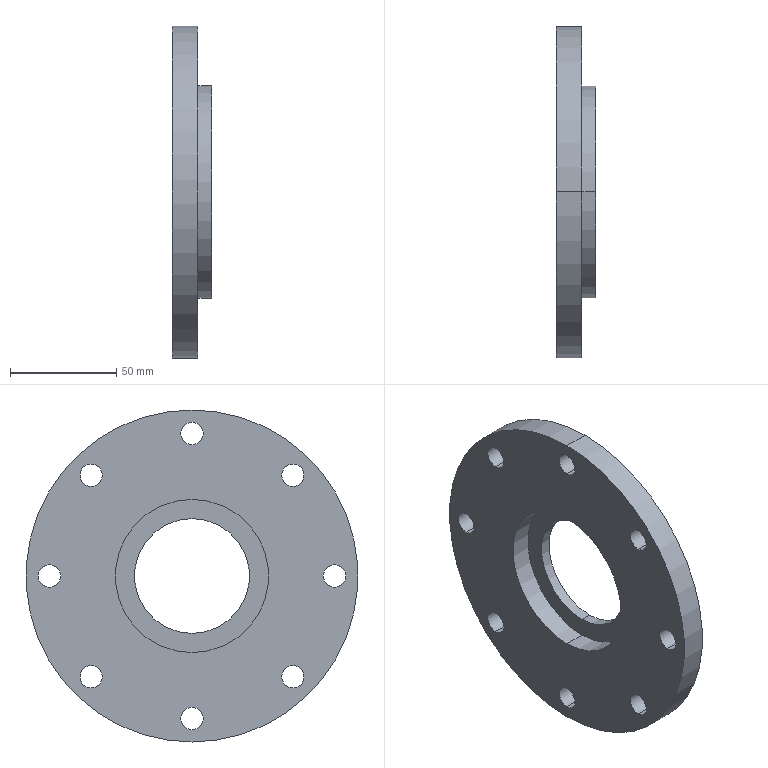Component | SolidWorks | UpperHousingAssembly-1_FlangeOnWormAxis-1 | 1 solid | 31 faces | box 18.5 x 156 x 156 mm | volume 196663 mm3 | cylinder 24 | plane 5 | cone 2 | commonest cylinder face diameters 10.5 x16 54 x2 100 x2 156 x2 72 x2
build123d program:
from build123d import *

# Parameters (mm, degrees)
SKETCH2_R          = 5.25
CUT_EXTRUDE1_DEPTH = 112.849
CIRPATTERN1_COUNT  = 8


with BuildPart() as part:
    # Sketch1 → Revolve1 (revolve)
    with BuildSketch(Plane.XY, mode=Mode.PRIVATE) as revolve1_sk:
        Polygon((0, 36), (0, 78), (12, 78), (12, 50), (18.5, 50), (18.5, 47), (15, 45), (15, 27), (10, 27), (10, 36), align=None)
    revolve(revolve1_sk.sketch.rotate(Axis((0, 0, 0), (1, 0, 0)), 90), axis=Axis((0, 0, 0), (1, 0, 0)))

    # Sketch2 → Cut-Extrude1 (cut, through all)
    with BuildSketch(Plane.ZY):
        with Locations((0, 67)):
            Circle(SKETCH2_R)
    cut_extrude1 = extrude(amount=-CUT_EXTRUDE1_DEPTH, mode=Mode.SUBTRACT)

    # CirPattern1: Cut-Extrude1 ×8 about axis
    cirpattern1_axis = Axis((0, 0, 0), (1, 0, 0))
    for i in range(1, CIRPATTERN1_COUNT):
        add(cut_extrude1.rotate(cirpattern1_axis, i * 360 / CIRPATTERN1_COUNT), mode=Mode.SUBTRACT)


solid = part.part

# Placed as in the assembly
solid = solid.moved(Location((719.83, 1408.591, 1694.217), (0, 0, 0)))
STEP:
#1=COLOUR_RGB('',0.7922,0.8196,0.9333);
#2=FILL_AREA_STYLE_COLOUR('',#1);
#3=FILL_AREA_STYLE('',(#2));
#4=SURFACE_STYLE_FILL_AREA(#3);
#5=SURFACE_SIDE_STYLE('',(#4));
#6=SURFACE_STYLE_USAGE(.BOTH.,#5);
#7=PRESENTATION_STYLE_ASSIGNMENT((#6));
#8=CARTESIAN_POINT('',(28.812,55.456,63.857));
#9=VERTEX_POINT('',#8);
#10=CARTESIAN_POINT('',(28.812,55.456,64.27));
#11=VERTEX_POINT('',#10);
#12=CARTESIAN_POINT('',(28.812,55.456,64.064));
#13=DIRECTION('',(-1.,0.,0.));
#14=DIRECTION('',(0.,0.,1.));
#15=AXIS2_PLACEMENT_3D('',#12,#13,#14);
#16=CIRCLE('',#15,0.2067);
#17=EDGE_CURVE('',#9,#11,#16,.T.);
#18=ORIENTED_EDGE('',*,*,#17,.F.);
#19=CARTESIAN_POINT('',(28.34,55.456,63.857));
#20=VERTEX_POINT('',#19);
#21=CARTESIAN_POINT('',(29.068,55.456,63.857));
#22=DIRECTION('',(-1.,0.,0.));
#23=VECTOR('',#22,39.37);
#24=LINE('',#21,#23);
#25=EDGE_CURVE('',#9,#20,#24,.T.);
#26=ORIENTED_EDGE('',*,*,#25,.T.);
#27=CARTESIAN_POINT('',(28.34,55.456,64.27));
#28=VERTEX_POINT('',#27);
#29=CARTESIAN_POINT('',(28.34,55.456,64.064));
#30=DIRECTION('',(-1.,0.,0.));
#31=DIRECTION('',(0.,1.,0.));
#32=AXIS2_PLACEMENT_3D('',#29,#30,#31);
#33=CIRCLE('',#32,0.2067);
#34=EDGE_CURVE('',#20,#28,#33,.T.);
#35=ORIENTED_EDGE('',*,*,#34,.T.);
#36=CARTESIAN_POINT('',(29.068,55.456,64.27));
#37=DIRECTION('',(-1.,0.,0.));
#38=VECTOR('',#37,39.37);
#39=LINE('',#36,#38);
#40=EDGE_CURVE('',#11,#28,#39,.T.);
#41=ORIENTED_EDGE('',*,*,#40,.F.);
#42=EDGE_LOOP('',(#18,#26,#35,#41));
#43=FACE_OUTER_BOUND('',#42,.T.);
#44=CARTESIAN_POINT('',(29.068,55.456,64.064));
#45=DIRECTION('',(-1.,0.,0.));
#46=DIRECTION('',(0.,0.,1.));
#47=AXIS2_PLACEMENT_3D('',#44,#45,#46);
#48=CYLINDRICAL_SURFACE('',#47,0.2067);
#49=ADVANCED_FACE('',(#43),#48,.F.);
#50=CARTESIAN_POINT('',(28.812,53.591,64.63));
#51=VERTEX_POINT('',#50);
#52=CARTESIAN_POINT('',(28.812,53.591,65.043));
#53=VERTEX_POINT('',#52);
#54=CARTESIAN_POINT('',(28.812,53.591,64.836));
#55=DIRECTION('',(-1.,0.,0.));
#56=DIRECTION('',(0.,0.,1.));
#57=AXIS2_PLACEMENT_3D('',#54,#55,#56);
#58=CIRCLE('',#57,0.2067);
#59=EDGE_CURVE('',#51,#53,#58,.T.);
#60=ORIENTED_EDGE('',*,*,#59,.F.);
#61=CARTESIAN_POINT('',(28.34,53.591,64.63));
#62=VERTEX_POINT('',#61);
#63=CARTESIAN_POINT('',(29.068,53.591,64.63));
#64=DIRECTION('',(-1.,0.,0.));
#65=VECTOR('',#64,39.37);
#66=LINE('',#63,#65);
#67=EDGE_CURVE('',#51,#62,#66,.T.);
#68=ORIENTED_EDGE('',*,*,#67,.T.);
#69=CARTESIAN_POINT('',(28.34,53.591,65.043));
#70=VERTEX_POINT('',#69);
#71=CARTESIAN_POINT('',(28.34,53.591,64.836));
#72=DIRECTION('',(-1.,0.,0.));
#73=DIRECTION('',(0.,0.7071,-0.7071));
#74=AXIS2_PLACEMENT_3D('',#71,#72,#73);
#75=CIRCLE('',#74,0.2067);
#76=EDGE_CURVE('',#62,#70,#75,.T.);
#77=ORIENTED_EDGE('',*,*,#76,.T.);
#78=CARTESIAN_POINT('',(29.068,53.591,65.043));
#79=DIRECTION('',(-1.,0.,0.));
#80=VECTOR('',#79,39.37);
#81=LINE('',#78,#80);
#82=EDGE_CURVE('',#53,#70,#81,.T.);
#83=ORIENTED_EDGE('',*,*,#82,.F.);
#84=EDGE_LOOP('',(#60,#68,#77,#83));
#85=FACE_OUTER_BOUND('',#84,.T.);
#86=CARTESIAN_POINT('',(29.068,53.591,64.836));
#87=DIRECTION('',(-1.,0.,0.));
#88=DIRECTION('',(0.,0.,1.));
#89=AXIS2_PLACEMENT_3D('',#86,#87,#88);
#90=CYLINDRICAL_SURFACE('',#89,0.2067);
#91=ADVANCED_FACE('',(#85),#90,.F.);
#92=CARTESIAN_POINT('',(28.812,52.819,66.495));
#93=VERTEX_POINT('',#92);
#94=CARTESIAN_POINT('',(28.812,52.819,66.908));
#95=VERTEX_POINT('',#94);
#96=CARTESIAN_POINT('',(28.812,52.819,66.701));
#97=DIRECTION('',(-1.,0.,0.));
#98=DIRECTION('',(0.,0.,1.));
#99=AXIS2_PLACEMENT_3D('',#96,#97,#98);
#100=CIRCLE('',#99,0.2067);
#101=EDGE_CURVE('',#93,#95,#100,.T.);
#102=ORIENTED_EDGE('',*,*,#101,.F.);
#103=CARTESIAN_POINT('',(28.34,52.819,66.495));
#104=VERTEX_POINT('',#103);
#105=CARTESIAN_POINT('',(29.068,52.819,66.495));
#106=DIRECTION('',(-1.,0.,0.));
#107=VECTOR('',#106,39.37);
#108=LINE('',#105,#107);
#109=EDGE_CURVE('',#93,#104,#108,.T.);
#110=ORIENTED_EDGE('',*,*,#109,.T.);
#111=CARTESIAN_POINT('',(28.34,52.819,66.908));
#112=VERTEX_POINT('',#111);
#113=CARTESIAN_POINT('',(28.34,52.819,66.701));
#114=DIRECTION('',(-1.,0.,0.));
#115=DIRECTION('',(0.,0.,-1.));
#116=AXIS2_PLACEMENT_3D('',#113,#114,#115);
#117=CIRCLE('',#116,0.2067);
#118=EDGE_CURVE('',#104,#112,#117,.T.);
#119=ORIENTED_EDGE('',*,*,#118,.T.);
#120=CARTESIAN_POINT('',(29.068,52.819,66.908));
#121=DIRECTION('',(-1.,0.,0.));
#122=VECTOR('',#121,39.37);
#123=LINE('',#120,#122);
#124=EDGE_CURVE('',#95,#112,#123,.T.);
#125=ORIENTED_EDGE('',*,*,#124,.F.);
#126=EDGE_LOOP('',(#102,#110,#119,#125));
#127=FACE_OUTER_BOUND('',#126,.T.);
#128=CARTESIAN_POINT('',(29.068,52.819,66.701));
#129=DIRECTION('',(-1.,0.,0.));
#130=DIRECTION('',(0.,0.,1.));
#131=AXIS2_PLACEMENT_3D('',#128,#129,#130);
#132=CYLINDRICAL_SURFACE('',#131,0.2067);
#133=ADVANCED_FACE('',(#127),#132,.F.);
#134=CARTESIAN_POINT('',(28.812,53.591,68.36));
#135=VERTEX_POINT('',#134);
#136=CARTESIAN_POINT('',(28.812,53.591,68.773));
#137=VERTEX_POINT('',#136);
#138=CARTESIAN_POINT('',(28.812,53.591,68.567));
#139=DIRECTION('',(-1.,0.,0.));
#140=DIRECTION('',(0.,0.,1.));
#141=AXIS2_PLACEMENT_3D('',#138,#139,#140);
#142=CIRCLE('',#141,0.2067);
#143=EDGE_CURVE('',#135,#137,#142,.T.);
#144=ORIENTED_EDGE('',*,*,#143,.F.);
#145=CARTESIAN_POINT('',(28.34,53.591,68.36));
#146=VERTEX_POINT('',#145);
#147=CARTESIAN_POINT('',(29.068,53.591,68.36));
#148=DIRECTION('',(-1.,0.,0.));
#149=VECTOR('',#148,39.37);
#150=LINE('',#147,#149);
#151=EDGE_CURVE('',#135,#146,#150,.T.);
#152=ORIENTED_EDGE('',*,*,#151,.T.);
#153=CARTESIAN_POINT('',(28.34,53.591,68.773));
#154=VERTEX_POINT('',#153);
#155=CARTESIAN_POINT('',(28.34,53.591,68.567));
#156=DIRECTION('',(-1.,0.,0.));
#157=DIRECTION('',(0.,-0.7071,-0.7071));
#158=AXIS2_PLACEMENT_3D('',#155,#156,#157);
#159=CIRCLE('',#158,0.2067);
#160=EDGE_CURVE('',#146,#154,#159,.T.);
#161=ORIENTED_EDGE('',*,*,#160,.T.);
#162=CARTESIAN_POINT('',(29.068,53.591,68.773));
#163=DIRECTION('',(-1.,0.,0.));
#164=VECTOR('',#163,39.37);
#165=LINE('',#162,#164);
#166=EDGE_CURVE('',#137,#154,#165,.T.);
#167=ORIENTED_EDGE('',*,*,#166,.F.);
#168=EDGE_LOOP('',(#144,#152,#161,#167));
#169=FACE_OUTER_BOUND('',#168,.T.);
#170=CARTESIAN_POINT('',(29.068,53.591,68.567));
#171=DIRECTION('',(-1.,0.,0.));
#172=DIRECTION('',(0.,0.,1.));
#173=AXIS2_PLACEMENT_3D('',#170,#171,#172);
#174=CYLINDRICAL_SURFACE('',#173,0.2067);
#175=ADVANCED_FACE('',(#169),#174,.F.);
#176=CARTESIAN_POINT('',(28.812,55.456,69.133));
#177=VERTEX_POINT('',#176);
#178=CARTESIAN_POINT('',(28.812,55.456,69.546));
#179=VERTEX_POINT('',#178);
#180=CARTESIAN_POINT('',(28.812,55.456,69.339));
#181=DIRECTION('',(-1.,0.,0.));
#182=DIRECTION('',(0.,0.,1.));
#183=AXIS2_PLACEMENT_3D('',#180,#181,#182);
#184=CIRCLE('',#183,0.2067);
#185=EDGE_CURVE('',#177,#179,#184,.T.);
#186=ORIENTED_EDGE('',*,*,#185,.F.);
#187=CARTESIAN_POINT('',(28.34,55.456,69.133));
#188=VERTEX_POINT('',#187);
#189=CARTESIAN_POINT('',(29.068,55.456,69.133));
#190=DIRECTION('',(-1.,0.,0.));
#191=VECTOR('',#190,39.37);
#192=LINE('',#189,#191);
#193=EDGE_CURVE('',#177,#188,#192,.T.);
#194=ORIENTED_EDGE('',*,*,#193,.T.);
#195=CARTESIAN_POINT('',(28.34,55.456,69.546));
#196=VERTEX_POINT('',#195);
#197=CARTESIAN_POINT('',(28.34,55.456,69.339));
#198=DIRECTION('',(-1.,0.,0.));
#199=DIRECTION('',(0.,-1.,0.));
#200=AXIS2_PLACEMENT_3D('',#197,#198,#199);
#201=CIRCLE('',#200,0.2067);
#202=EDGE_CURVE('',#188,#196,#201,.T.);
#203=ORIENTED_EDGE('',*,*,#202,.T.);
#204=CARTESIAN_POINT('',(29.068,55.456,69.546));
#205=DIRECTION('',(-1.,0.,0.));
#206=VECTOR('',#205,39.37);
#207=LINE('',#204,#206);
#208=EDGE_CURVE('',#179,#196,#207,.T.);
#209=ORIENTED_EDGE('',*,*,#208,.F.);
#210=EDGE_LOOP('',(#186,#194,#203,#209));
#211=FACE_OUTER_BOUND('',#210,.T.);
#212=CARTESIAN_POINT('',(29.068,55.456,69.339));
#213=DIRECTION('',(-1.,0.,0.));
#214=DIRECTION('',(0.,0.,1.));
#215=AXIS2_PLACEMENT_3D('',#212,#213,#214);
#216=CYLINDRICAL_SURFACE('',#215,0.2067);
#217=ADVANCED_FACE('',(#211),#216,.F.);
#218=CARTESIAN_POINT('',(28.812,57.322,68.36));
#219=VERTEX_POINT('',#218);
#220=CARTESIAN_POINT('',(28.812,57.322,68.773));
#221=VERTEX_POINT('',#220);
#222=CARTESIAN_POINT('',(28.812,57.322,68.567));
#223=DIRECTION('',(-1.,0.,0.));
#224=DIRECTION('',(0.,0.,1.));
#225=AXIS2_PLACEMENT_3D('',#222,#223,#224);
#226=CIRCLE('',#225,0.2067);
#227=EDGE_CURVE('',#219,#221,#226,.T.);
#228=ORIENTED_EDGE('',*,*,#227,.F.);
#229=CARTESIAN_POINT('',(28.34,57.322,68.36));
#230=VERTEX_POINT('',#229);
#231=CARTESIAN_POINT('',(29.068,57.322,68.36));
#232=DIRECTION('',(-1.,0.,0.));
#233=VECTOR('',#232,39.37);
#234=LINE('',#231,#233);
#235=EDGE_CURVE('',#219,#230,#234,.T.);
#236=ORIENTED_EDGE('',*,*,#235,.T.);
#237=CARTESIAN_POINT('',(28.34,57.322,68.773));
#238=VERTEX_POINT('',#237);
#239=CARTESIAN_POINT('',(28.34,57.322,68.567));
#240=DIRECTION('',(-1.,0.,0.));
#241=DIRECTION('',(0.,-0.7071,0.7071));
#242=AXIS2_PLACEMENT_3D('',#239,#240,#241);
#243=CIRCLE('',#242,0.2067);
#244=EDGE_CURVE('',#230,#238,#243,.T.);
#245=ORIENTED_EDGE('',*,*,#244,.T.);
#246=CARTESIAN_POINT('',(29.068,57.322,68.773));
#247=DIRECTION('',(-1.,0.,0.));
#248=VECTOR('',#247,39.37);
#249=LINE('',#246,#248);
#250=EDGE_CURVE('',#221,#238,#249,.T.);
#251=ORIENTED_EDGE('',*,*,#250,.F.);
#252=EDGE_LOOP('',(#228,#236,#245,#251));
#253=FACE_OUTER_BOUND('',#252,.T.);
#254=CARTESIAN_POINT('',(29.068,57.322,68.567));
#255=DIRECTION('',(-1.,0.,0.));
#256=DIRECTION('',(0.,0.,1.));
#257=AXIS2_PLACEMENT_3D('',#254,#255,#256);
#258=CYLINDRICAL_SURFACE('',#257,0.2067);
#259=ADVANCED_FACE('',(#253),#258,.F.);
#260=CARTESIAN_POINT('',(28.812,57.322,64.63));
#261=VERTEX_POINT('',#260);
#262=CARTESIAN_POINT('',(28.812,57.322,65.043));
#263=VERTEX_POINT('',#262);
#264=CARTESIAN_POINT('',(28.812,57.322,64.836));
#265=DIRECTION('',(-1.,0.,0.));
#266=DIRECTION('',(0.,0.,1.));
#267=AXIS2_PLACEMENT_3D('',#264,#265,#266);
#268=CIRCLE('',#267,0.2067);
#269=EDGE_CURVE('',#261,#263,#268,.T.);
#270=ORIENTED_EDGE('',*,*,#269,.F.);
#271=CARTESIAN_POINT('',(28.34,57.322,64.63));
#272=VERTEX_POINT('',#271);
#273=CARTESIAN_POINT('',(29.068,57.322,64.63));
#274=DIRECTION('',(-1.,0.,0.));
#275=VECTOR('',#274,39.37);
#276=LINE('',#273,#275);
#277=EDGE_CURVE('',#261,#272,#276,.T.);
#278=ORIENTED_EDGE('',*,*,#277,.T.);
#279=CARTESIAN_POINT('',(28.34,57.322,65.043));
#280=VERTEX_POINT('',#279);
#281=CARTESIAN_POINT('',(28.34,57.322,64.836));
#282=DIRECTION('',(-1.,0.,0.));
#283=DIRECTION('',(0.,0.7071,0.7071));
#284=AXIS2_PLACEMENT_3D('',#281,#282,#283);
#285=CIRCLE('',#284,0.2067);
#286=EDGE_CURVE('',#272,#280,#285,.T.);
#287=ORIENTED_EDGE('',*,*,#286,.T.);
#288=CARTESIAN_POINT('',(29.068,57.322,65.043));
#289=DIRECTION('',(-1.,0.,0.));
#290=VECTOR('',#289,39.37);
#291=LINE('',#288,#290);
#292=EDGE_CURVE('',#263,#280,#291,.T.);
#293=ORIENTED_EDGE('',*,*,#292,.F.);
#294=EDGE_LOOP('',(#270,#278,#287,#293));
#295=FACE_OUTER_BOUND('',#294,.T.);
#296=CARTESIAN_POINT('',(29.068,57.322,64.836));
#297=DIRECTION('',(-1.,0.,0.));
#298=DIRECTION('',(0.,0.,1.));
#299=AXIS2_PLACEMENT_3D('',#296,#297,#298);
#300=CYLINDRICAL_SURFACE('',#299,0.2067);
#301=ADVANCED_FACE('',(#295),#300,.F.);
#302=CARTESIAN_POINT('',(28.812,58.094,66.495));
#303=VERTEX_POINT('',#302);
#304=CARTESIAN_POINT('',(28.812,58.094,66.908));
#305=VERTEX_POINT('',#304);
#306=CARTESIAN_POINT('',(28.812,58.094,66.701));
#307=DIRECTION('',(-1.,0.,0.));
#308=DIRECTION('',(0.,0.,1.));
#309=AXIS2_PLACEMENT_3D('',#306,#307,#308);
#310=CIRCLE('',#309,0.2067);
#311=EDGE_CURVE('',#303,#305,#310,.T.);
#312=ORIENTED_EDGE('',*,*,#311,.F.);
#313=CARTESIAN_POINT('',(28.34,58.094,66.495));
#314=VERTEX_POINT('',#313);
#315=CARTESIAN_POINT('',(29.068,58.094,66.495));
#316=DIRECTION('',(-1.,0.,0.));
#317=VECTOR('',#316,39.37);
#318=LINE('',#315,#317);
#319=EDGE_CURVE('',#303,#314,#318,.T.);
#320=ORIENTED_EDGE('',*,*,#319,.T.);
#321=CARTESIAN_POINT('',(28.34,58.094,66.908));
#322=VERTEX_POINT('',#321);
#323=CARTESIAN_POINT('',(28.34,58.094,66.701));
#324=DIRECTION('',(-1.,0.,0.));
#325=DIRECTION('',(0.,0.,1.));
#326=AXIS2_PLACEMENT_3D('',#323,#324,#325);
#327=CIRCLE('',#326,0.2067);
#328=EDGE_CURVE('',#314,#322,#327,.T.);
#329=ORIENTED_EDGE('',*,*,#328,.T.);
#330=CARTESIAN_POINT('',(29.068,58.094,66.908));
#331=DIRECTION('',(-1.,0.,0.));
#332=VECTOR('',#331,39.37);
#333=LINE('',#330,#332);
#334=EDGE_CURVE('',#305,#322,#333,.T.);
#335=ORIENTED_EDGE('',*,*,#334,.F.);
#336=EDGE_LOOP('',(#312,#320,#329,#335));
#337=FACE_OUTER_BOUND('',#336,.T.);
#338=CARTESIAN_POINT('',(29.068,58.094,66.701));
#339=DIRECTION('',(-1.,0.,0.));
#340=DIRECTION('',(0.,0.,1.));
#341=AXIS2_PLACEMENT_3D('',#338,#339,#340);
#342=CYLINDRICAL_SURFACE('',#341,0.2067);
#343=ADVANCED_FACE('',(#337),#342,.F.);
#344=CARTESIAN_POINT('',(28.93,55.456,65.638));
#345=VERTEX_POINT('',#344);
#346=CARTESIAN_POINT('',(28.93,55.456,67.764));
#347=VERTEX_POINT('',#346);
#348=CARTESIAN_POINT('',(28.93,55.456,66.701));
#349=DIRECTION('',(-1.,0.,0.));
#350=DIRECTION('',(0.,0.,1.));
#351=AXIS2_PLACEMENT_3D('',#348,#349,#350);
#352=CIRCLE('',#351,1.063);
#353=EDGE_CURVE('',#345,#347,#352,.T.);
#354=ORIENTED_EDGE('',*,*,#353,.F.);
#355=CARTESIAN_POINT('',(28.733,55.456,65.638));
#356=VERTEX_POINT('',#355);
#357=CARTESIAN_POINT('',(28.34,55.456,65.638));
#358=DIRECTION('',(-1.,0.,0.));
#359=VECTOR('',#358,39.37);
#360=LINE('',#357,#359);
#361=EDGE_CURVE('',#345,#356,#360,.T.);
#362=ORIENTED_EDGE('',*,*,#361,.T.);
#363=CARTESIAN_POINT('',(28.733,55.456,67.764));
#364=VERTEX_POINT('',#363);
#365=CARTESIAN_POINT('',(28.733,55.456,66.701));
#366=DIRECTION('',(-1.,0.,0.));
#367=DIRECTION('',(0.,0.,1.));
#368=AXIS2_PLACEMENT_3D('',#365,#366,#367);
#369=CIRCLE('',#368,1.063);
#370=EDGE_CURVE('',#356,#364,#369,.T.);
#371=ORIENTED_EDGE('',*,*,#370,.T.);
#372=CARTESIAN_POINT('',(28.34,55.456,67.764));
#373=DIRECTION('',(-1.,0.,0.));
#374=VECTOR('',#373,39.37);
#375=LINE('',#372,#374);
#376=EDGE_CURVE('',#347,#364,#375,.T.);
#377=ORIENTED_EDGE('',*,*,#376,.F.);
#378=EDGE_LOOP('',(#354,#362,#371,#377));
#379=FACE_OUTER_BOUND('',#378,.T.);
#380=CARTESIAN_POINT('',(28.34,55.456,66.701));
#381=DIRECTION('',(-1.,0.,0.));
#382=DIRECTION('',(0.,0.,1.));
#383=AXIS2_PLACEMENT_3D('',#380,#381,#382);
#384=CYLINDRICAL_SURFACE('',#383,1.063);
#385=ADVANCED_FACE('',(#379),#384,.F.);
#386=CARTESIAN_POINT('',(28.93,55.456,64.93));
#387=VERTEX_POINT('',#386);
#388=CARTESIAN_POINT('',(28.93,55.456,68.473));
#389=VERTEX_POINT('',#388);
#390=CARTESIAN_POINT('',(28.93,55.456,66.701));
#391=DIRECTION('',(-1.,0.,0.));
#392=DIRECTION('',(0.,0.,1.));
#393=AXIS2_PLACEMENT_3D('',#390,#391,#392);
#394=CIRCLE('',#393,1.772);
#395=EDGE_CURVE('',#387,#389,#394,.T.);
#396=ORIENTED_EDGE('',*,*,#395,.T.);
#397=CARTESIAN_POINT('',(29.068,55.456,68.552));
#398=VERTEX_POINT('',#397);
#399=CARTESIAN_POINT('',(28.93,55.456,68.473));
#400=DIRECTION('',(0.8682,0.,0.4961));
#401=VECTOR('',#400,39.37);
#402=LINE('',#399,#401);
#403=EDGE_CURVE('',#389,#398,#402,.T.);
#404=ORIENTED_EDGE('',*,*,#403,.T.);
#405=CARTESIAN_POINT('',(29.068,55.456,64.851));
#406=VERTEX_POINT('',#405);
#407=CARTESIAN_POINT('',(29.068,55.456,66.701));
#408=DIRECTION('',(-1.,0.,0.));
#409=DIRECTION('',(0.,0.,1.));
#410=AXIS2_PLACEMENT_3D('',#407,#408,#409);
#411=CIRCLE('',#410,1.85);
#412=EDGE_CURVE('',#406,#398,#411,.T.);
#413=ORIENTED_EDGE('',*,*,#412,.F.);
#414=CARTESIAN_POINT('',(28.93,55.456,64.93));
#415=DIRECTION('',(0.8682,0.,-0.4961));
#416=VECTOR('',#415,39.37);
#417=LINE('',#414,#416);
#418=EDGE_CURVE('',#387,#406,#417,.T.);
#419=ORIENTED_EDGE('',*,*,#418,.F.);
#420=EDGE_LOOP('',(#396,#404,#413,#419));
#421=FACE_OUTER_BOUND('',#420,.T.);
#422=CARTESIAN_POINT('',(28.93,55.456,66.701));
#423=DIRECTION('',(1.,0.,0.));
#424=DIRECTION('',(0.,0.,-1.));
#425=AXIS2_PLACEMENT_3D('',#422,#423,#424);
#426=CONICAL_SURFACE('',#425,1.772,0.5191);
#427=ADVANCED_FACE('',(#421),#426,.F.);
#428=CARTESIAN_POINT('',(29.068,55.456,68.67));
#429=VERTEX_POINT('',#428);
#430=CARTESIAN_POINT('',(29.068,55.456,64.733));
#431=VERTEX_POINT('',#430);
#432=CARTESIAN_POINT('',(29.068,55.456,66.701));
#433=DIRECTION('',(-1.,0.,0.));
#434=DIRECTION('',(0.,0.,1.));
#435=AXIS2_PLACEMENT_3D('',#432,#433,#434);
#436=CIRCLE('',#435,1.969);
#437=EDGE_CURVE('',#429,#431,#436,.T.);
#438=ORIENTED_EDGE('',*,*,#437,.T.);
#439=CARTESIAN_POINT('',(28.812,55.456,64.733));
#440=VERTEX_POINT('',#439);
#441=CARTESIAN_POINT('',(28.34,55.456,64.733));
#442=DIRECTION('',(-1.,0.,0.));
#443=VECTOR('',#442,39.37);
#444=LINE('',#441,#443);
#445=EDGE_CURVE('',#431,#440,#444,.T.);
#446=ORIENTED_EDGE('',*,*,#445,.T.);
#447=CARTESIAN_POINT('',(28.812,55.456,68.67));
#448=VERTEX_POINT('',#447);
#449=CARTESIAN_POINT('',(28.812,55.456,66.701));
#450=DIRECTION('',(-1.,0.,0.));
#451=DIRECTION('',(0.,0.,1.));
#452=AXIS2_PLACEMENT_3D('',#449,#450,#451);
#453=CIRCLE('',#452,1.969);
#454=EDGE_CURVE('',#448,#440,#453,.T.);
#455=ORIENTED_EDGE('',*,*,#454,.F.);
#456=CARTESIAN_POINT('',(28.34,55.456,68.67));
#457=DIRECTION('',(-1.,0.,0.));
#458=VECTOR('',#457,39.37);
#459=LINE('',#456,#458);
#460=EDGE_CURVE('',#429,#448,#459,.T.);
#461=ORIENTED_EDGE('',*,*,#460,.F.);
#462=EDGE_LOOP('',(#438,#446,#455,#461));
#463=FACE_OUTER_BOUND('',#462,.T.);
#464=CARTESIAN_POINT('',(28.34,55.456,66.701));
#465=DIRECTION('',(-1.,0.,0.));
#466=DIRECTION('',(0.,0.,1.));
#467=AXIS2_PLACEMENT_3D('',#464,#465,#466);
#468=CYLINDRICAL_SURFACE('',#467,1.969);
#469=ADVANCED_FACE('',(#463),#468,.T.);
#470=CARTESIAN_POINT('',(28.812,55.456,69.772));
#471=VERTEX_POINT('',#470);
#472=CARTESIAN_POINT('',(28.812,55.456,63.631));
#473=VERTEX_POINT('',#472);
#474=CARTESIAN_POINT('',(28.812,55.456,66.701));
#475=DIRECTION('',(-1.,0.,0.));
#476=DIRECTION('',(0.,0.,1.));
#477=AXIS2_PLACEMENT_3D('',#474,#475,#476);
#478=CIRCLE('',#477,3.071);
#479=EDGE_CURVE('',#471,#473,#478,.T.);
#480=ORIENTED_EDGE('',*,*,#479,.T.);
#481=CARTESIAN_POINT('',(28.34,55.456,63.631));
#482=VERTEX_POINT('',#481);
#483=CARTESIAN_POINT('',(28.34,55.456,63.631));
#484=DIRECTION('',(-1.,0.,0.));
#485=VECTOR('',#484,39.37);
#486=LINE('',#483,#485);
#487=EDGE_CURVE('',#473,#482,#486,.T.);
#488=ORIENTED_EDGE('',*,*,#487,.T.);
#489=CARTESIAN_POINT('',(28.34,55.456,69.772));
#490=VERTEX_POINT('',#489);
#491=CARTESIAN_POINT('',(28.34,55.456,66.701));
#492=DIRECTION('',(-1.,0.,0.));
#493=DIRECTION('',(0.,0.,1.));
#494=AXIS2_PLACEMENT_3D('',#491,#492,#493);
#495=CIRCLE('',#494,3.071);
#496=EDGE_CURVE('',#490,#482,#495,.T.);
#497=ORIENTED_EDGE('',*,*,#496,.F.);
#498=CARTESIAN_POINT('',(28.34,55.456,69.772));
#499=DIRECTION('',(-1.,0.,0.));
#500=VECTOR('',#499,39.37);
#501=LINE('',#498,#500);
#502=EDGE_CURVE('',#471,#490,#501,.T.);
#503=ORIENTED_EDGE('',*,*,#502,.F.);
#504=EDGE_LOOP('',(#480,#488,#497,#503));
#505=FACE_OUTER_BOUND('',#504,.T.);
#506=CARTESIAN_POINT('',(28.34,55.456,66.701));
#507=DIRECTION('',(-1.,0.,0.));
#508=DIRECTION('',(0.,0.,1.));
#509=AXIS2_PLACEMENT_3D('',#506,#507,#508);
#510=CYLINDRICAL_SURFACE('',#509,3.071);
#511=ADVANCED_FACE('',(#505),#510,.T.);
#512=CARTESIAN_POINT('',(28.733,55.456,65.284));
#513=VERTEX_POINT('',#512);
#514=CARTESIAN_POINT('',(28.733,55.456,68.119));
#515=VERTEX_POINT('',#514);
#516=CARTESIAN_POINT('',(28.733,55.456,66.701));
#517=DIRECTION('',(-1.,0.,0.));
#518=DIRECTION('',(0.,0.,1.));
#519=AXIS2_PLACEMENT_3D('',#516,#517,#518);
#520=CIRCLE('',#519,1.417);
#521=EDGE_CURVE('',#513,#515,#520,.T.);
#522=ORIENTED_EDGE('',*,*,#521,.F.);
#523=CARTESIAN_POINT('',(28.34,55.456,65.284));
#524=VERTEX_POINT('',#523);
#525=CARTESIAN_POINT('',(28.34,55.456,65.284));
#526=DIRECTION('',(-1.,0.,0.));
#527=VECTOR('',#526,39.37);
#528=LINE('',#525,#527);
#529=EDGE_CURVE('',#513,#524,#528,.T.);
#530=ORIENTED_EDGE('',*,*,#529,.T.);
#531=CARTESIAN_POINT('',(28.34,55.456,68.119));
#532=VERTEX_POINT('',#531);
#533=CARTESIAN_POINT('',(28.34,55.456,66.701));
#534=DIRECTION('',(-1.,0.,0.));
#535=DIRECTION('',(0.,0.,1.));
#536=AXIS2_PLACEMENT_3D('',#533,#534,#535);
#537=CIRCLE('',#536,1.417);
#538=EDGE_CURVE('',#524,#532,#537,.T.);
#539=ORIENTED_EDGE('',*,*,#538,.T.);
#540=CARTESIAN_POINT('',(28.34,55.456,68.119));
#541=DIRECTION('',(-1.,0.,0.));
#542=VECTOR('',#541,39.37);
#543=LINE('',#540,#542);
#544=EDGE_CURVE('',#515,#532,#543,.T.);
#545=ORIENTED_EDGE('',*,*,#544,.F.);
#546=EDGE_LOOP('',(#522,#530,#539,#545));
#547=FACE_OUTER_BOUND('',#546,.T.);
#548=CARTESIAN_POINT('',(28.34,55.456,66.701));
#549=DIRECTION('',(-1.,0.,0.));
#550=DIRECTION('',(0.,0.,1.));
#551=AXIS2_PLACEMENT_3D('',#548,#549,#550);
#552=CYLINDRICAL_SURFACE('',#551,1.417);
#553=ADVANCED_FACE('',(#547),#552,.F.);
#554=ORIENTED_EDGE('',*,*,#529,.F.);
#555=CARTESIAN_POINT('',(28.733,55.456,66.701));
#556=DIRECTION('',(-1.,0.,0.));
#557=DIRECTION('',(0.,0.,1.));
#558=AXIS2_PLACEMENT_3D('',#555,#556,#557);
#559=CIRCLE('',#558,1.417);
#560=EDGE_CURVE('',#515,#513,#559,.T.);
#561=ORIENTED_EDGE('',*,*,#560,.F.);
#562=ORIENTED_EDGE('',*,*,#544,.T.);
#563=CARTESIAN_POINT('',(28.34,55.456,66.701));
#564=DIRECTION('',(-1.,0.,0.));
#565=DIRECTION('',(0.,0.,1.));
#566=AXIS2_PLACEMENT_3D('',#563,#564,#565);
#567=CIRCLE('',#566,1.417);
#568=EDGE_CURVE('',#532,#524,#567,.T.);
#569=ORIENTED_EDGE('',*,*,#568,.T.);
#570=EDGE_LOOP('',(#554,#561,#562,#569));
#571=FACE_OUTER_BOUND('',#570,.T.);
#572=CARTESIAN_POINT('',(28.34,55.456,66.701));
#573=DIRECTION('',(-1.,0.,0.));
#574=DIRECTION('',(0.,0.,1.));
#575=AXIS2_PLACEMENT_3D('',#572,#573,#574);
#576=CYLINDRICAL_SURFACE('',#575,1.417);
#577=ADVANCED_FACE('',(#571),#576,.F.);
#578=CARTESIAN_POINT('',(28.34,55.456,64.064));
#579=DIRECTION('',(-1.,0.,0.));
#580=DIRECTION('',(0.,1.,0.));
#581=AXIS2_PLACEMENT_3D('',#578,#579,#580);
#582=CIRCLE('',#581,0.2067);
#583=EDGE_CURVE('',#28,#20,#582,.T.);
#584=ORIENTED_EDGE('',*,*,#583,.F.);
#585=ORIENTED_EDGE('',*,*,#34,.F.);
#586=EDGE_LOOP('',(#584,#585));
#587=FACE_BOUND('',#586,.T.);
#588=CARTESIAN_POINT('',(28.34,53.591,64.836));
#589=DIRECTION('',(-1.,0.,0.));
#590=DIRECTION('',(0.,0.7071,-0.7071));
#591=AXIS2_PLACEMENT_3D('',#588,#589,#590);
#592=CIRCLE('',#591,0.2067);
#593=EDGE_CURVE('',#70,#62,#592,.T.);
#594=ORIENTED_EDGE('',*,*,#593,.F.);
#595=ORIENTED_EDGE('',*,*,#76,.F.);
#596=EDGE_LOOP('',(#594,#595));
#597=FACE_BOUND('',#596,.T.);
#598=CARTESIAN_POINT('',(28.34,52.819,66.701));
#599=DIRECTION('',(-1.,0.,0.));
#600=DIRECTION('',(0.,0.,-1.));
#601=AXIS2_PLACEMENT_3D('',#598,#599,#600);
#602=CIRCLE('',#601,0.2067);
#603=EDGE_CURVE('',#112,#104,#602,.T.);
#604=ORIENTED_EDGE('',*,*,#603,.F.);
#605=ORIENTED_EDGE('',*,*,#118,.F.);
#606=EDGE_LOOP('',(#604,#605));
#607=FACE_BOUND('',#606,.T.);
#608=CARTESIAN_POINT('',(28.34,53.591,68.567));
#609=DIRECTION('',(-1.,0.,0.));
#610=DIRECTION('',(0.,-0.7071,-0.7071));
#611=AXIS2_PLACEMENT_3D('',#608,#609,#610);
#612=CIRCLE('',#611,0.2067);
#613=EDGE_CURVE('',#154,#146,#612,.T.);
#614=ORIENTED_EDGE('',*,*,#613,.F.);
#615=ORIENTED_EDGE('',*,*,#160,.F.);
#616=EDGE_LOOP('',(#614,#615));
#617=FACE_BOUND('',#616,.T.);
#618=CARTESIAN_POINT('',(28.34,55.456,69.339));
#619=DIRECTION('',(-1.,0.,0.));
#620=DIRECTION('',(0.,-1.,0.));
#621=AXIS2_PLACEMENT_3D('',#618,#619,#620);
#622=CIRCLE('',#621,0.2067);
#623=EDGE_CURVE('',#196,#188,#622,.T.);
#624=ORIENTED_EDGE('',*,*,#623,.F.);
#625=ORIENTED_EDGE('',*,*,#202,.F.);
#626=EDGE_LOOP('',(#624,#625));
#627=FACE_BOUND('',#626,.T.);
#628=CARTESIAN_POINT('',(28.34,57.322,68.567));
#629=DIRECTION('',(-1.,0.,0.));
#630=DIRECTION('',(0.,-0.7071,0.7071));
#631=AXIS2_PLACEMENT_3D('',#628,#629,#630);
#632=CIRCLE('',#631,0.2067);
#633=EDGE_CURVE('',#238,#230,#632,.T.);
#634=ORIENTED_EDGE('',*,*,#633,.F.);
#635=ORIENTED_EDGE('',*,*,#244,.F.);
#636=EDGE_LOOP('',(#634,#635));
#637=FACE_BOUND('',#636,.T.);
#638=CARTESIAN_POINT('',(28.34,57.322,64.836));
#639=DIRECTION('',(-1.,0.,0.));
#640=DIRECTION('',(0.,0.7071,0.7071));
#641=AXIS2_PLACEMENT_3D('',#638,#639,#640);
#642=CIRCLE('',#641,0.2067);
#643=EDGE_CURVE('',#280,#272,#642,.T.);
#644=ORIENTED_EDGE('',*,*,#643,.F.);
#645=ORIENTED_EDGE('',*,*,#286,.F.);
#646=EDGE_LOOP('',(#644,#645));
#647=FACE_BOUND('',#646,.T.);
#648=CARTESIAN_POINT('',(28.34,58.094,66.701));
#649=DIRECTION('',(-1.,0.,0.));
#650=DIRECTION('',(0.,0.,1.));
#651=AXIS2_PLACEMENT_3D('',#648,#649,#650);
#652=CIRCLE('',#651,0.2067);
#653=EDGE_CURVE('',#322,#314,#652,.T.);
#654=ORIENTED_EDGE('',*,*,#653,.F.);
#655=ORIENTED_EDGE('',*,*,#328,.F.);
#656=EDGE_LOOP('',(#654,#655));
#657=FACE_BOUND('',#656,.T.);
#658=ORIENTED_EDGE('',*,*,#568,.F.);
#659=ORIENTED_EDGE('',*,*,#538,.F.);
#660=EDGE_LOOP('',(#658,#659));
#661=FACE_BOUND('',#660,.T.);
#662=ORIENTED_EDGE('',*,*,#496,.T.);
#663=CARTESIAN_POINT('',(28.34,55.456,66.701));
#664=DIRECTION('',(-1.,0.,0.));
#665=DIRECTION('',(0.,0.,1.));
#666=AXIS2_PLACEMENT_3D('',#663,#664,#665);
#667=CIRCLE('',#666,3.071);
#668=EDGE_CURVE('',#482,#490,#667,.T.);
#669=ORIENTED_EDGE('',*,*,#668,.T.);
#670=EDGE_LOOP('',(#662,#669));
#671=FACE_OUTER_BOUND('',#670,.T.);
#672=CARTESIAN_POINT('',(28.34,56.874,66.701));
#673=DIRECTION('',(1.,0.,0.));
#674=DIRECTION('',(0.,0.,-1.));
#675=AXIS2_PLACEMENT_3D('',#672,#673,#674);
#676=PLANE('',#675);
#677=ADVANCED_FACE('',(#587,#597,#607,#617,#627,#637,#647,#657,#661,#671),#676,.F.);
#678=ORIENTED_EDGE('',*,*,#487,.F.);
#679=CARTESIAN_POINT('',(28.812,55.456,66.701));
#680=DIRECTION('',(-1.,0.,0.));
#681=DIRECTION('',(0.,0.,1.));
#682=AXIS2_PLACEMENT_3D('',#679,#680,#681);
#683=CIRCLE('',#682,3.071);
#684=EDGE_CURVE('',#473,#471,#683,.T.);
#685=ORIENTED_EDGE('',*,*,#684,.T.);
#686=ORIENTED_EDGE('',*,*,#502,.T.);
#687=ORIENTED_EDGE('',*,*,#668,.F.);
#688=EDGE_LOOP('',(#678,#685,#686,#687));
#689=FACE_OUTER_BOUND('',#688,.T.);
#690=CARTESIAN_POINT('',(28.34,55.456,66.701));
#691=DIRECTION('',(-1.,0.,0.));
#692=DIRECTION('',(0.,0.,1.));
#693=AXIS2_PLACEMENT_3D('',#690,#691,#692);
#694=CYLINDRICAL_SURFACE('',#693,3.071);
#695=ADVANCED_FACE('',(#689),#694,.T.);
#696=CARTESIAN_POINT('',(28.812,55.456,64.064));
#697=DIRECTION('',(-1.,0.,0.));
#698=DIRECTION('',(0.,0.,1.));
#699=AXIS2_PLACEMENT_3D('',#696,#697,#698);
#700=CIRCLE('',#699,0.2067);
#701=EDGE_CURVE('',#11,#9,#700,.T.);
#702=ORIENTED_EDGE('',*,*,#701,.T.);
#703=ORIENTED_EDGE('',*,*,#17,.T.);
#704=EDGE_LOOP('',(#702,#703));
#705=FACE_BOUND('',#704,.T.);
#706=CARTESIAN_POINT('',(28.812,53.591,64.836));
#707=DIRECTION('',(-1.,0.,0.));
#708=DIRECTION('',(0.,0.,1.));
#709=AXIS2_PLACEMENT_3D('',#706,#707,#708);
#710=CIRCLE('',#709,0.2067);
#711=EDGE_CURVE('',#53,#51,#710,.T.);
#712=ORIENTED_EDGE('',*,*,#711,.T.);
#713=ORIENTED_EDGE('',*,*,#59,.T.);
#714=EDGE_LOOP('',(#712,#713));
#715=FACE_BOUND('',#714,.T.);
#716=CARTESIAN_POINT('',(28.812,52.819,66.701));
#717=DIRECTION('',(-1.,0.,0.));
#718=DIRECTION('',(0.,0.,1.));
#719=AXIS2_PLACEMENT_3D('',#716,#717,#718);
#720=CIRCLE('',#719,0.2067);
#721=EDGE_CURVE('',#95,#93,#720,.T.);
#722=ORIENTED_EDGE('',*,*,#721,.T.);
#723=ORIENTED_EDGE('',*,*,#101,.T.);
#724=EDGE_LOOP('',(#722,#723));
#725=FACE_BOUND('',#724,.T.);
#726=CARTESIAN_POINT('',(28.812,53.591,68.567));
#727=DIRECTION('',(-1.,0.,0.));
#728=DIRECTION('',(0.,0.,1.));
#729=AXIS2_PLACEMENT_3D('',#726,#727,#728);
#730=CIRCLE('',#729,0.2067);
#731=EDGE_CURVE('',#137,#135,#730,.T.);
#732=ORIENTED_EDGE('',*,*,#731,.T.);
#733=ORIENTED_EDGE('',*,*,#143,.T.);
#734=EDGE_LOOP('',(#732,#733));
#735=FACE_BOUND('',#734,.T.);
#736=CARTESIAN_POINT('',(28.812,55.456,69.339));
#737=DIRECTION('',(-1.,0.,0.));
#738=DIRECTION('',(0.,0.,1.));
#739=AXIS2_PLACEMENT_3D('',#736,#737,#738);
#740=CIRCLE('',#739,0.2067);
#741=EDGE_CURVE('',#179,#177,#740,.T.);
#742=ORIENTED_EDGE('',*,*,#741,.T.);
#743=ORIENTED_EDGE('',*,*,#185,.T.);
#744=EDGE_LOOP('',(#742,#743));
#745=FACE_BOUND('',#744,.T.);
#746=CARTESIAN_POINT('',(28.812,57.322,68.567));
#747=DIRECTION('',(-1.,0.,0.));
#748=DIRECTION('',(0.,0.,1.));
#749=AXIS2_PLACEMENT_3D('',#746,#747,#748);
#750=CIRCLE('',#749,0.2067);
#751=EDGE_CURVE('',#221,#219,#750,.T.);
#752=ORIENTED_EDGE('',*,*,#751,.T.);
#753=ORIENTED_EDGE('',*,*,#227,.T.);
#754=EDGE_LOOP('',(#752,#753));
#755=FACE_BOUND('',#754,.T.);
#756=CARTESIAN_POINT('',(28.812,57.322,64.836));
#757=DIRECTION('',(-1.,0.,0.));
#758=DIRECTION('',(0.,0.,1.));
#759=AXIS2_PLACEMENT_3D('',#756,#757,#758);
#760=CIRCLE('',#759,0.2067);
#761=EDGE_CURVE('',#263,#261,#760,.T.);
#762=ORIENTED_EDGE('',*,*,#761,.T.);
#763=ORIENTED_EDGE('',*,*,#269,.T.);
#764=EDGE_LOOP('',(#762,#763));
#765=FACE_BOUND('',#764,.T.);
#766=CARTESIAN_POINT('',(28.812,58.094,66.701));
#767=DIRECTION('',(-1.,0.,0.));
#768=DIRECTION('',(0.,0.,1.));
#769=AXIS2_PLACEMENT_3D('',#766,#767,#768);
#770=CIRCLE('',#769,0.2067);
#771=EDGE_CURVE('',#305,#303,#770,.T.);
#772=ORIENTED_EDGE('',*,*,#771,.T.);
#773=ORIENTED_EDGE('',*,*,#311,.T.);
#774=EDGE_LOOP('',(#772,#773));
#775=FACE_BOUND('',#774,.T.);
#776=ORIENTED_EDGE('',*,*,#479,.F.);
#777=ORIENTED_EDGE('',*,*,#684,.F.);
#778=EDGE_LOOP('',(#776,#777));
#779=FACE_OUTER_BOUND('',#778,.T.);
#780=ORIENTED_EDGE('',*,*,#454,.T.);
#781=CARTESIAN_POINT('',(28.812,55.456,66.701));
#782=DIRECTION('',(-1.,0.,0.));
#783=DIRECTION('',(0.,0.,1.));
#784=AXIS2_PLACEMENT_3D('',#781,#782,#783);
#785=CIRCLE('',#784,1.969);
#786=EDGE_CURVE('',#440,#448,#785,.T.);
#787=ORIENTED_EDGE('',*,*,#786,.T.);
#788=EDGE_LOOP('',(#780,#787));
#789=FACE_BOUND('',#788,.T.);
#790=CARTESIAN_POINT('',(28.812,58.527,66.701));
#791=DIRECTION('',(-1.,0.,0.));
#792=DIRECTION('',(0.,0.,1.));
#793=AXIS2_PLACEMENT_3D('',#790,#791,#792);
#794=PLANE('',#793);
#795=ADVANCED_FACE('',(#705,#715,#725,#735,#745,#755,#765,#775,#779,#789),#794,.F.);
#796=ORIENTED_EDGE('',*,*,#445,.F.);
#797=CARTESIAN_POINT('',(29.068,55.456,66.701));
#798=DIRECTION('',(-1.,0.,0.));
#799=DIRECTION('',(0.,0.,1.));
#800=AXIS2_PLACEMENT_3D('',#797,#798,#799);
#801=CIRCLE('',#800,1.969);
#802=EDGE_CURVE('',#431,#429,#801,.T.);
#803=ORIENTED_EDGE('',*,*,#802,.T.);
#804=ORIENTED_EDGE('',*,*,#460,.T.);
#805=ORIENTED_EDGE('',*,*,#786,.F.);
#806=EDGE_LOOP('',(#796,#803,#804,#805));
#807=FACE_OUTER_BOUND('',#806,.T.);
#808=CARTESIAN_POINT('',(28.34,55.456,66.701));
#809=DIRECTION('',(-1.,0.,0.));
#810=DIRECTION('',(0.,0.,1.));
#811=AXIS2_PLACEMENT_3D('',#808,#809,#810);
#812=CYLINDRICAL_SURFACE('',#811,1.969);
#813=ADVANCED_FACE('',(#807),#812,.T.);
#814=ORIENTED_EDGE('',*,*,#437,.F.);
#815=ORIENTED_EDGE('',*,*,#802,.F.);
#816=EDGE_LOOP('',(#814,#815));
#817=FACE_OUTER_BOUND('',#816,.T.);
#818=ORIENTED_EDGE('',*,*,#412,.T.);
#819=CARTESIAN_POINT('',(29.068,55.456,66.701));
#820=DIRECTION('',(-1.,0.,0.));
#821=DIRECTION('',(0.,0.,1.));
#822=AXIS2_PLACEMENT_3D('',#819,#820,#821);
#823=CIRCLE('',#822,1.85);
#824=EDGE_CURVE('',#398,#406,#823,.T.);
#825=ORIENTED_EDGE('',*,*,#824,.T.);
#826=EDGE_LOOP('',(#818,#825));
#827=FACE_BOUND('',#826,.T.);
#828=CARTESIAN_POINT('',(29.068,57.425,66.701));
#829=DIRECTION('',(-1.,0.,0.));
#830=DIRECTION('',(0.,0.,1.));
#831=AXIS2_PLACEMENT_3D('',#828,#829,#830);
#832=PLANE('',#831);
#833=ADVANCED_FACE('',(#817,#827),#832,.F.);
#834=ORIENTED_EDGE('',*,*,#403,.F.);
#835=CARTESIAN_POINT('',(28.93,55.456,66.701));
#836=DIRECTION('',(-1.,0.,0.));
#837=DIRECTION('',(0.,0.,1.));
#838=AXIS2_PLACEMENT_3D('',#835,#836,#837);
#839=CIRCLE('',#838,1.772);
#840=EDGE_CURVE('',#389,#387,#839,.T.);
#841=ORIENTED_EDGE('',*,*,#840,.T.);
#842=ORIENTED_EDGE('',*,*,#418,.T.);
#843=ORIENTED_EDGE('',*,*,#824,.F.);
#844=EDGE_LOOP('',(#834,#841,#842,#843));
#845=FACE_OUTER_BOUND('',#844,.T.);
#846=CARTESIAN_POINT('',(28.93,55.456,66.701));
#847=DIRECTION('',(1.,0.,0.));
#848=DIRECTION('',(0.,0.,-1.));
#849=AXIS2_PLACEMENT_3D('',#846,#847,#848);
#850=CONICAL_SURFACE('',#849,1.772,0.5191);
#851=ADVANCED_FACE('',(#845),#850,.F.);
#852=ORIENTED_EDGE('',*,*,#395,.F.);
#853=ORIENTED_EDGE('',*,*,#840,.F.);
#854=EDGE_LOOP('',(#852,#853));
#855=FACE_OUTER_BOUND('',#854,.T.);
#856=CARTESIAN_POINT('',(28.93,55.456,66.701));
#857=DIRECTION('',(-1.,0.,0.));
#858=DIRECTION('',(0.,0.,1.));
#859=AXIS2_PLACEMENT_3D('',#856,#857,#858);
#860=CIRCLE('',#859,1.063);
#861=EDGE_CURVE('',#347,#345,#860,.T.);
#862=ORIENTED_EDGE('',*,*,#861,.T.);
#863=ORIENTED_EDGE('',*,*,#353,.T.);
#864=EDGE_LOOP('',(#862,#863));
#865=FACE_BOUND('',#864,.T.);
#866=CARTESIAN_POINT('',(28.93,57.228,66.701));
#867=DIRECTION('',(-1.,0.,0.));
#868=DIRECTION('',(0.,0.,1.));
#869=AXIS2_PLACEMENT_3D('',#866,#867,#868);
#870=PLANE('',#869);
#871=ADVANCED_FACE('',(#855,#865),#870,.F.);
#872=ORIENTED_EDGE('',*,*,#361,.F.);
#873=ORIENTED_EDGE('',*,*,#861,.F.);
#874=ORIENTED_EDGE('',*,*,#376,.T.);
#875=CARTESIAN_POINT('',(28.733,55.456,66.701));
#876=DIRECTION('',(-1.,0.,0.));
#877=DIRECTION('',(0.,0.,1.));
#878=AXIS2_PLACEMENT_3D('',#875,#876,#877);
#879=CIRCLE('',#878,1.063);
#880=EDGE_CURVE('',#364,#356,#879,.T.);
#881=ORIENTED_EDGE('',*,*,#880,.T.);
#882=EDGE_LOOP('',(#872,#873,#874,#881));
#883=FACE_OUTER_BOUND('',#882,.T.);
#884=CARTESIAN_POINT('',(28.34,55.456,66.701));
#885=DIRECTION('',(-1.,0.,0.));
#886=DIRECTION('',(0.,0.,1.));
#887=AXIS2_PLACEMENT_3D('',#884,#885,#886);
#888=CYLINDRICAL_SURFACE('',#887,1.063);
#889=ADVANCED_FACE('',(#883),#888,.F.);
#890=ORIENTED_EDGE('',*,*,#880,.F.);
#891=ORIENTED_EDGE('',*,*,#370,.F.);
#892=EDGE_LOOP('',(#890,#891));
#893=FACE_BOUND('',#892,.T.);
#894=ORIENTED_EDGE('',*,*,#560,.T.);
#895=ORIENTED_EDGE('',*,*,#521,.T.);
#896=EDGE_LOOP('',(#894,#895));
#897=FACE_OUTER_BOUND('',#896,.T.);
#898=CARTESIAN_POINT('',(28.733,56.519,66.701));
#899=DIRECTION('',(1.,0.,0.));
#900=DIRECTION('',(0.,0.,-1.));
#901=AXIS2_PLACEMENT_3D('',#898,#899,#900);
#902=PLANE('',#901);
#903=ADVANCED_FACE('',(#893,#897),#902,.F.);
#904=ORIENTED_EDGE('',*,*,#319,.F.);
#905=ORIENTED_EDGE('',*,*,#771,.F.);
#906=ORIENTED_EDGE('',*,*,#334,.T.);
#907=ORIENTED_EDGE('',*,*,#653,.T.);
#908=EDGE_LOOP('',(#904,#905,#906,#907));
#909=FACE_OUTER_BOUND('',#908,.T.);
#910=CARTESIAN_POINT('',(29.068,58.094,66.701));
#911=DIRECTION('',(-1.,0.,0.));
#912=DIRECTION('',(0.,0.,1.));
#913=AXIS2_PLACEMENT_3D('',#910,#911,#912);
#914=CYLINDRICAL_SURFACE('',#913,0.2067);
#915=ADVANCED_FACE('',(#909),#914,.F.);
#916=ORIENTED_EDGE('',*,*,#277,.F.);
#917=ORIENTED_EDGE('',*,*,#761,.F.);
#918=ORIENTED_EDGE('',*,*,#292,.T.);
#919=ORIENTED_EDGE('',*,*,#643,.T.);
#920=EDGE_LOOP('',(#916,#917,#918,#919));
#921=FACE_OUTER_BOUND('',#920,.T.);
#922=CARTESIAN_POINT('',(29.068,57.322,64.836));
#923=DIRECTION('',(-1.,0.,0.));
#924=DIRECTION('',(0.,0.,1.));
#925=AXIS2_PLACEMENT_3D('',#922,#923,#924);
#926=CYLINDRICAL_SURFACE('',#925,0.2067);
#927=ADVANCED_FACE('',(#921),#926,.F.);
#928=ORIENTED_EDGE('',*,*,#235,.F.);
#929=ORIENTED_EDGE('',*,*,#751,.F.);
#930=ORIENTED_EDGE('',*,*,#250,.T.);
#931=ORIENTED_EDGE('',*,*,#633,.T.);
#932=EDGE_LOOP('',(#928,#929,#930,#931));
#933=FACE_OUTER_BOUND('',#932,.T.);
#934=CARTESIAN_POINT('',(29.068,57.322,68.567));
#935=DIRECTION('',(-1.,0.,0.));
#936=DIRECTION('',(0.,0.,1.));
#937=AXIS2_PLACEMENT_3D('',#934,#935,#936);
#938=CYLINDRICAL_SURFACE('',#937,0.2067);
#939=ADVANCED_FACE('',(#933),#938,.F.);
#940=ORIENTED_EDGE('',*,*,#193,.F.);
#941=ORIENTED_EDGE('',*,*,#741,.F.);
#942=ORIENTED_EDGE('',*,*,#208,.T.);
#943=ORIENTED_EDGE('',*,*,#623,.T.);
#944=EDGE_LOOP('',(#940,#941,#942,#943));
#945=FACE_OUTER_BOUND('',#944,.T.);
#946=CARTESIAN_POINT('',(29.068,55.456,69.339));
#947=DIRECTION('',(-1.,0.,0.));
#948=DIRECTION('',(0.,0.,1.));
#949=AXIS2_PLACEMENT_3D('',#946,#947,#948);
#950=CYLINDRICAL_SURFACE('',#949,0.2067);
#951=ADVANCED_FACE('',(#945),#950,.F.);
#952=ORIENTED_EDGE('',*,*,#151,.F.);
#953=ORIENTED_EDGE('',*,*,#731,.F.);
#954=ORIENTED_EDGE('',*,*,#166,.T.);
#955=ORIENTED_EDGE('',*,*,#613,.T.);
#956=EDGE_LOOP('',(#952,#953,#954,#955));
#957=FACE_OUTER_BOUND('',#956,.T.);
#958=CARTESIAN_POINT('',(29.068,53.591,68.567));
#959=DIRECTION('',(-1.,0.,0.));
#960=DIRECTION('',(0.,0.,1.));
#961=AXIS2_PLACEMENT_3D('',#958,#959,#960);
#962=CYLINDRICAL_SURFACE('',#961,0.2067);
#963=ADVANCED_FACE('',(#957),#962,.F.);
#964=ORIENTED_EDGE('',*,*,#109,.F.);
#965=ORIENTED_EDGE('',*,*,#721,.F.);
#966=ORIENTED_EDGE('',*,*,#124,.T.);
#967=ORIENTED_EDGE('',*,*,#603,.T.);
#968=EDGE_LOOP('',(#964,#965,#966,#967));
#969=FACE_OUTER_BOUND('',#968,.T.);
#970=CARTESIAN_POINT('',(29.068,52.819,66.701));
#971=DIRECTION('',(-1.,0.,0.));
#972=DIRECTION('',(0.,0.,1.));
#973=AXIS2_PLACEMENT_3D('',#970,#971,#972);
#974=CYLINDRICAL_SURFACE('',#973,0.2067);
#975=ADVANCED_FACE('',(#969),#974,.F.);
#976=ORIENTED_EDGE('',*,*,#67,.F.);
#977=ORIENTED_EDGE('',*,*,#711,.F.);
#978=ORIENTED_EDGE('',*,*,#82,.T.);
#979=ORIENTED_EDGE('',*,*,#593,.T.);
#980=EDGE_LOOP('',(#976,#977,#978,#979));
#981=FACE_OUTER_BOUND('',#980,.T.);
#982=CARTESIAN_POINT('',(29.068,53.591,64.836));
#983=DIRECTION('',(-1.,0.,0.));
#984=DIRECTION('',(0.,0.,1.));
#985=AXIS2_PLACEMENT_3D('',#982,#983,#984);
#986=CYLINDRICAL_SURFACE('',#985,0.2067);
#987=ADVANCED_FACE('',(#981),#986,.F.);
#988=ORIENTED_EDGE('',*,*,#25,.F.);
#989=ORIENTED_EDGE('',*,*,#701,.F.);
#990=ORIENTED_EDGE('',*,*,#40,.T.);
#991=ORIENTED_EDGE('',*,*,#583,.T.);
#992=EDGE_LOOP('',(#988,#989,#990,#991));
#993=FACE_OUTER_BOUND('',#992,.T.);
#994=CARTESIAN_POINT('',(29.068,55.456,64.064));
#995=DIRECTION('',(-1.,0.,0.));
#996=DIRECTION('',(0.,0.,1.));
#997=AXIS2_PLACEMENT_3D('',#994,#995,#996);
#998=CYLINDRICAL_SURFACE('',#997,0.2067);
#999=ADVANCED_FACE('',(#993),#998,.F.);
#1000=CLOSED_SHELL('',(#49,#91,#133,#175,#217,#259,#301,#343,#385,#427,#469,#511,#553,#577,#677,#695,#795,#813,#833,#851,#871,#889,#903,#915,#927,#939,#951,#963,#975,#987,#999));
#1001=MANIFOLD_SOLID_BREP('',#1000);
#1002=STYLED_ITEM('',(#7),#1001);
#1003=(LENGTH_UNIT()NAMED_UNIT(*)SI_UNIT($,.METRE.));
#1004=LENGTH_MEASURE_WITH_UNIT(LENGTH_MEASURE(0.0254),#1003);
#1005=DIMENSIONAL_EXPONENTS(1.,0.,0.,0.,0.,0.,0.);
#1006=(CONVERSION_BASED_UNIT('',#1004)LENGTH_UNIT()NAMED_UNIT(#1005));
#1007=UNCERTAINTY_MEASURE_WITH_UNIT(LENGTH_MEASURE(0.00001),#1006,'','');
#1008=(NAMED_UNIT(*)PLANE_ANGLE_UNIT()SI_UNIT($,.RADIAN.));
#1009=(NAMED_UNIT(*)SI_UNIT($,.STERADIAN.)SOLID_ANGLE_UNIT());
#1010=(GEOMETRIC_REPRESENTATION_CONTEXT(3)GLOBAL_UNCERTAINTY_ASSIGNED_CONTEXT((#1007))GLOBAL_UNIT_ASSIGNED_CONTEXT((#1006,#1008,#1009))REPRESENTATION_CONTEXT('',''));
#1011=MECHANICAL_DESIGN_GEOMETRIC_PRESENTATION_REPRESENTATION('',(#1002),#1010);
#1012=CARTESIAN_POINT('',(0.,0.,0.));
#1013=DIRECTION('',(0.,0.,1.));
#1014=DIRECTION('',(1.,0.,0.));
#1015=AXIS2_PLACEMENT_3D('',#1012,#1013,#1014);
#1016=(LENGTH_UNIT()NAMED_UNIT(*)SI_UNIT($,.METRE.));
#1017=LENGTH_MEASURE_WITH_UNIT(LENGTH_MEASURE(0.0254),#1016);
#1018=DIMENSIONAL_EXPONENTS(1.,0.,0.,0.,0.,0.,0.);
#1019=(CONVERSION_BASED_UNIT('',#1017)LENGTH_UNIT()NAMED_UNIT(#1018));
#1020=UNCERTAINTY_MEASURE_WITH_UNIT(LENGTH_MEASURE(0.00001),#1019,'','');
#1021=(NAMED_UNIT(*)PLANE_ANGLE_UNIT()SI_UNIT($,.RADIAN.));
#1022=(NAMED_UNIT(*)SI_UNIT($,.STERADIAN.)SOLID_ANGLE_UNIT());
#1023=(GEOMETRIC_REPRESENTATION_CONTEXT(3)GLOBAL_UNCERTAINTY_ASSIGNED_CONTEXT((#1020))GLOBAL_UNIT_ASSIGNED_CONTEXT((#1019,#1021,#1022))REPRESENTATION_CONTEXT('',''));
#1024=ADVANCED_BREP_SHAPE_REPRESENTATION('',(#1001,#1015),#1023);
#1025=PRESENTATION_LAYER_ASSIGNMENT('','',(#1002));